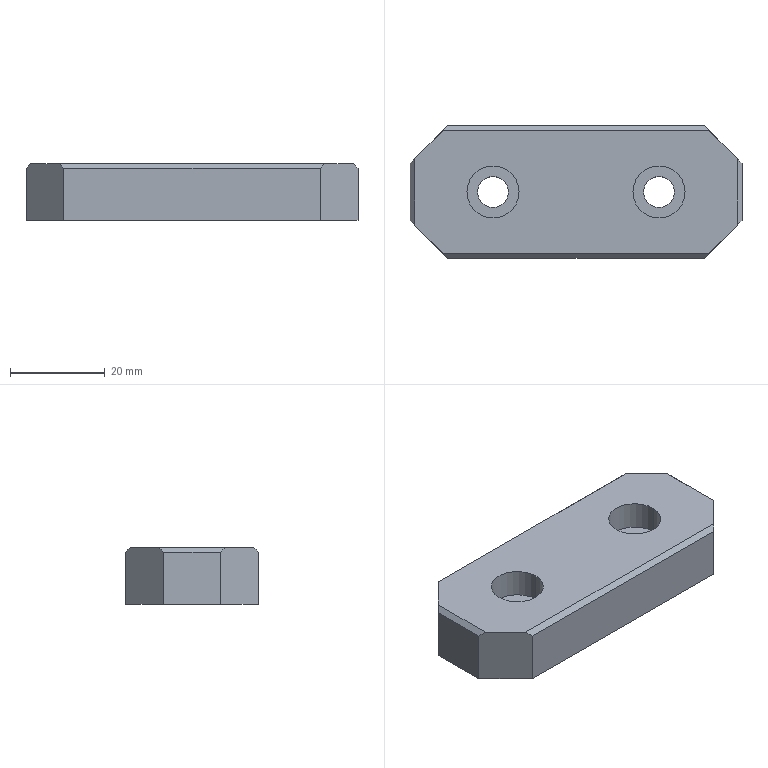Component | SolidWorks | DZ.KX.203-TC1505-30-09-01-05-05-1 | 1 solid | 24 faces | box 70 x 28 x 12 mm | volume 20378 mm3 | plane 16 | cylinder 8 | commonest cylinder face diameters 11 x4 6.5 x4 | material Plain Carbon Steel
build123d program:
from build123d import *

# Parameters (mm, degrees)
SKETCH1_W                                         = 70
SKETCH1_H                                         = 28
BOSS_EXTRUDE1_DEPTH                               = 12
HOLE_SIZE_ACCORDING_TO_HEXAGON_SOCKET_D           = 6.5
HOLE_SIZE_ACCORDING_TO_HEXAGON_SOCKET_CBORE_D     = 11
HOLE_SIZE_ACCORDING_TO_HEXAGON_SOCKET_CBORE_DEPTH = 6
CHAMFER2_SIZE                                     = 8
CHAMFER3_SIZE                                     = 1


with BuildPart() as part:
    # Sketch1 → Boss-Extrude1 (new body)
    with BuildSketch(Plane(origin=(0, 0, 0), x_dir=(0, 0, -1), z_dir=(1, 0, 0))):
        Rectangle(SKETCH1_W, SKETCH1_H)
    extrude(amount=BOSS_EXTRUDE1_DEPTH)

    # Hole Size _according to_ Hexagon Socket (through all)
    with Locations(Plane.ZY):
        with Locations((-17.5, 0), (17.5, 0)):
            CounterBoreHole(HOLE_SIZE_ACCORDING_TO_HEXAGON_SOCKET_D / 2, HOLE_SIZE_ACCORDING_TO_HEXAGON_SOCKET_CBORE_D / 2, HOLE_SIZE_ACCORDING_TO_HEXAGON_SOCKET_CBORE_DEPTH)

    # Chamfer2
    chamfer2_edges = [part.edges().sort_by_distance(p)[0] for p in [
        (6, 14, 35),
        (6, 14, -35),
        (6, -14, -35),
        (6, -14, 35),
    ]]
    chamfer(chamfer2_edges, length=CHAMFER2_SIZE)

    # Chamfer3
    chamfer3_edges = [part.edges().sort_by_distance(p)[0] for p in [
        (0, 0, 35),
        (0, 14, 0),
        (0, 0, -35),
        (0, -14, 0),
    ]]
    chamfer(chamfer3_edges, length=CHAMFER3_SIZE)


solid = part.part

# Placed as in the assembly
solid = solid.moved(Location((294.5, -610.807, 225.06), (0, 90, 0)))
STEP:
#1=COLOUR_RGB('',0.7922,0.8196,0.9333);
#2=FILL_AREA_STYLE_COLOUR('',#1);
#3=FILL_AREA_STYLE('',(#2));
#4=SURFACE_STYLE_FILL_AREA(#3);
#5=SURFACE_SIDE_STYLE('',(#4));
#6=SURFACE_STYLE_USAGE(.BOTH.,#5);
#7=PRESENTATION_STYLE_ASSIGNMENT((#6));
#8=CARTESIAN_POINT('',(10.689,-24.048,8.624));
#9=VERTEX_POINT('',#8);
#10=CARTESIAN_POINT('',(11.122,-24.048,8.624));
#11=VERTEX_POINT('',#10);
#12=CARTESIAN_POINT('',(10.906,-24.048,8.624));
#13=DIRECTION('',(0.,-0.,1.));
#14=DIRECTION('',(1.,0.,0.));
#15=AXIS2_PLACEMENT_3D('',#12,#13,#14);
#16=CIRCLE('',#15,0.2165);
#17=EDGE_CURVE('',#9,#11,#16,.T.);
#18=ORIENTED_EDGE('',*,*,#17,.F.);
#19=CARTESIAN_POINT('',(10.689,-24.048,8.861));
#20=VERTEX_POINT('',#19);
#21=CARTESIAN_POINT('',(10.689,-24.048,8.861));
#22=DIRECTION('',(0.,-0.,1.));
#23=VECTOR('',#22,39.37);
#24=LINE('',#21,#23);
#25=EDGE_CURVE('',#9,#20,#24,.T.);
#26=ORIENTED_EDGE('',*,*,#25,.T.);
#27=CARTESIAN_POINT('',(11.122,-24.048,8.861));
#28=VERTEX_POINT('',#27);
#29=CARTESIAN_POINT('',(10.906,-24.048,8.861));
#30=DIRECTION('',(0.,-0.,1.));
#31=DIRECTION('',(1.,0.,0.));
#32=AXIS2_PLACEMENT_3D('',#29,#30,#31);
#33=CIRCLE('',#32,0.2165);
#34=EDGE_CURVE('',#20,#28,#33,.T.);
#35=ORIENTED_EDGE('',*,*,#34,.T.);
#36=CARTESIAN_POINT('',(11.122,-24.048,8.861));
#37=DIRECTION('',(0.,-0.,1.));
#38=VECTOR('',#37,39.37);
#39=LINE('',#36,#38);
#40=EDGE_CURVE('',#11,#28,#39,.T.);
#41=ORIENTED_EDGE('',*,*,#40,.F.);
#42=EDGE_LOOP('',(#18,#26,#35,#41));
#43=FACE_OUTER_BOUND('',#42,.T.);
#44=CARTESIAN_POINT('',(10.906,-24.048,8.861));
#45=DIRECTION('',(0.,-0.,1.));
#46=DIRECTION('',(1.,0.,0.));
#47=AXIS2_PLACEMENT_3D('',#44,#45,#46);
#48=CYLINDRICAL_SURFACE('',#47,0.2165);
#49=ADVANCED_FACE('',(#43),#48,.F.);
#50=CARTESIAN_POINT('',(10.778,-24.048,8.388));
#51=VERTEX_POINT('',#50);
#52=CARTESIAN_POINT('',(11.033,-24.048,8.388));
#53=VERTEX_POINT('',#52);
#54=CARTESIAN_POINT('',(10.906,-24.048,8.388));
#55=DIRECTION('',(0.,-0.,1.));
#56=DIRECTION('',(1.,0.,0.));
#57=AXIS2_PLACEMENT_3D('',#54,#55,#56);
#58=CIRCLE('',#57,0.128);
#59=EDGE_CURVE('',#51,#53,#58,.T.);
#60=ORIENTED_EDGE('',*,*,#59,.F.);
#61=CARTESIAN_POINT('',(10.778,-24.048,8.624));
#62=VERTEX_POINT('',#61);
#63=CARTESIAN_POINT('',(10.778,-24.048,8.861));
#64=DIRECTION('',(0.,-0.,1.));
#65=VECTOR('',#64,39.37);
#66=LINE('',#63,#65);
#67=EDGE_CURVE('',#51,#62,#66,.T.);
#68=ORIENTED_EDGE('',*,*,#67,.T.);
#69=CARTESIAN_POINT('',(11.033,-24.048,8.624));
#70=VERTEX_POINT('',#69);
#71=CARTESIAN_POINT('',(10.906,-24.048,8.624));
#72=DIRECTION('',(0.,-0.,1.));
#73=DIRECTION('',(1.,0.,0.));
#74=AXIS2_PLACEMENT_3D('',#71,#72,#73);
#75=CIRCLE('',#74,0.128);
#76=EDGE_CURVE('',#62,#70,#75,.T.);
#77=ORIENTED_EDGE('',*,*,#76,.T.);
#78=CARTESIAN_POINT('',(11.033,-24.048,8.861));
#79=DIRECTION('',(0.,-0.,1.));
#80=VECTOR('',#79,39.37);
#81=LINE('',#78,#80);
#82=EDGE_CURVE('',#53,#70,#81,.T.);
#83=ORIENTED_EDGE('',*,*,#82,.F.);
#84=EDGE_LOOP('',(#60,#68,#77,#83));
#85=FACE_OUTER_BOUND('',#84,.T.);
#86=CARTESIAN_POINT('',(10.906,-24.048,8.861));
#87=DIRECTION('',(0.,-0.,1.));
#88=DIRECTION('',(1.,0.,0.));
#89=AXIS2_PLACEMENT_3D('',#86,#87,#88);
#90=CYLINDRICAL_SURFACE('',#89,0.128);
#91=ADVANCED_FACE('',(#85),#90,.F.);
#92=CARTESIAN_POINT('',(12.067,-24.048,8.624));
#93=VERTEX_POINT('',#92);
#94=CARTESIAN_POINT('',(12.5,-24.048,8.624));
#95=VERTEX_POINT('',#94);
#96=CARTESIAN_POINT('',(12.283,-24.048,8.624));
#97=DIRECTION('',(0.,-0.,1.));
#98=DIRECTION('',(1.,0.,0.));
#99=AXIS2_PLACEMENT_3D('',#96,#97,#98);
#100=CIRCLE('',#99,0.2165);
#101=EDGE_CURVE('',#93,#95,#100,.T.);
#102=ORIENTED_EDGE('',*,*,#101,.F.);
#103=CARTESIAN_POINT('',(12.067,-24.048,8.861));
#104=VERTEX_POINT('',#103);
#105=CARTESIAN_POINT('',(12.067,-24.048,8.861));
#106=DIRECTION('',(0.,-0.,1.));
#107=VECTOR('',#106,39.37);
#108=LINE('',#105,#107);
#109=EDGE_CURVE('',#93,#104,#108,.T.);
#110=ORIENTED_EDGE('',*,*,#109,.T.);
#111=CARTESIAN_POINT('',(12.5,-24.048,8.861));
#112=VERTEX_POINT('',#111);
#113=CARTESIAN_POINT('',(12.283,-24.048,8.861));
#114=DIRECTION('',(0.,-0.,1.));
#115=DIRECTION('',(1.,0.,0.));
#116=AXIS2_PLACEMENT_3D('',#113,#114,#115);
#117=CIRCLE('',#116,0.2165);
#118=EDGE_CURVE('',#104,#112,#117,.T.);
#119=ORIENTED_EDGE('',*,*,#118,.T.);
#120=CARTESIAN_POINT('',(12.5,-24.048,8.861));
#121=DIRECTION('',(0.,-0.,1.));
#122=VECTOR('',#121,39.37);
#123=LINE('',#120,#122);
#124=EDGE_CURVE('',#95,#112,#123,.T.);
#125=ORIENTED_EDGE('',*,*,#124,.F.);
#126=EDGE_LOOP('',(#102,#110,#119,#125));
#127=FACE_OUTER_BOUND('',#126,.T.);
#128=CARTESIAN_POINT('',(12.283,-24.048,8.861));
#129=DIRECTION('',(0.,-0.,1.));
#130=DIRECTION('',(1.,0.,0.));
#131=AXIS2_PLACEMENT_3D('',#128,#129,#130);
#132=CYLINDRICAL_SURFACE('',#131,0.2165);
#133=ADVANCED_FACE('',(#127),#132,.F.);
#134=CARTESIAN_POINT('',(12.156,-24.048,8.388));
#135=VERTEX_POINT('',#134);
#136=CARTESIAN_POINT('',(12.411,-24.048,8.388));
#137=VERTEX_POINT('',#136);
#138=CARTESIAN_POINT('',(12.283,-24.048,8.388));
#139=DIRECTION('',(0.,-0.,1.));
#140=DIRECTION('',(1.,0.,0.));
#141=AXIS2_PLACEMENT_3D('',#138,#139,#140);
#142=CIRCLE('',#141,0.128);
#143=EDGE_CURVE('',#135,#137,#142,.T.);
#144=ORIENTED_EDGE('',*,*,#143,.F.);
#145=CARTESIAN_POINT('',(12.156,-24.048,8.624));
#146=VERTEX_POINT('',#145);
#147=CARTESIAN_POINT('',(12.156,-24.048,8.861));
#148=DIRECTION('',(0.,-0.,1.));
#149=VECTOR('',#148,39.37);
#150=LINE('',#147,#149);
#151=EDGE_CURVE('',#135,#146,#150,.T.);
#152=ORIENTED_EDGE('',*,*,#151,.T.);
#153=CARTESIAN_POINT('',(12.411,-24.048,8.624));
#154=VERTEX_POINT('',#153);
#155=CARTESIAN_POINT('',(12.283,-24.048,8.624));
#156=DIRECTION('',(0.,-0.,1.));
#157=DIRECTION('',(1.,0.,0.));
#158=AXIS2_PLACEMENT_3D('',#155,#156,#157);
#159=CIRCLE('',#158,0.128);
#160=EDGE_CURVE('',#146,#154,#159,.T.);
#161=ORIENTED_EDGE('',*,*,#160,.T.);
#162=CARTESIAN_POINT('',(12.411,-24.048,8.861));
#163=DIRECTION('',(0.,-0.,1.));
#164=VECTOR('',#163,39.37);
#165=LINE('',#162,#164);
#166=EDGE_CURVE('',#137,#154,#165,.T.);
#167=ORIENTED_EDGE('',*,*,#166,.F.);
#168=EDGE_LOOP('',(#144,#152,#161,#167));
#169=FACE_OUTER_BOUND('',#168,.T.);
#170=CARTESIAN_POINT('',(12.283,-24.048,8.861));
#171=DIRECTION('',(0.,-0.,1.));
#172=DIRECTION('',(1.,0.,0.));
#173=AXIS2_PLACEMENT_3D('',#170,#171,#172);
#174=CYLINDRICAL_SURFACE('',#173,0.128);
#175=ADVANCED_FACE('',(#169),#174,.F.);
#176=CARTESIAN_POINT('',(12.972,-23.811,8.388));
#177=VERTEX_POINT('',#176);
#178=CARTESIAN_POINT('',(12.972,-23.811,8.821));
#179=VERTEX_POINT('',#178);
#180=CARTESIAN_POINT('',(12.972,-23.811,8.388));
#181=DIRECTION('',(0.,-0.,1.));
#182=VECTOR('',#181,39.37);
#183=LINE('',#180,#182);
#184=EDGE_CURVE('',#177,#179,#183,.T.);
#185=ORIENTED_EDGE('',*,*,#184,.T.);
#186=CARTESIAN_POINT('',(12.972,-24.284,8.821));
#187=VERTEX_POINT('',#186);
#188=CARTESIAN_POINT('',(12.972,-24.599,8.821));
#189=DIRECTION('',(-0.,-1.,-0.));
#190=VECTOR('',#189,39.37);
#191=LINE('',#188,#190);
#192=EDGE_CURVE('',#179,#187,#191,.T.);
#193=ORIENTED_EDGE('',*,*,#192,.T.);
#194=CARTESIAN_POINT('',(12.972,-24.284,8.388));
#195=VERTEX_POINT('',#194);
#196=CARTESIAN_POINT('',(12.972,-24.284,8.388));
#197=DIRECTION('',(-0.,0.,-1.));
#198=VECTOR('',#197,39.37);
#199=LINE('',#196,#198);
#200=EDGE_CURVE('',#187,#195,#199,.T.);
#201=ORIENTED_EDGE('',*,*,#200,.T.);
#202=CARTESIAN_POINT('',(12.972,-24.599,8.388));
#203=DIRECTION('',(-0.,-1.,-0.));
#204=VECTOR('',#203,39.37);
#205=LINE('',#202,#204);
#206=EDGE_CURVE('',#177,#195,#205,.T.);
#207=ORIENTED_EDGE('',*,*,#206,.F.);
#208=EDGE_LOOP('',(#185,#193,#201,#207));
#209=FACE_OUTER_BOUND('',#208,.T.);
#210=CARTESIAN_POINT('',(12.972,-24.599,8.388));
#211=DIRECTION('',(-1.,0.,0.));
#212=DIRECTION('',(0.,-0.,1.));
#213=AXIS2_PLACEMENT_3D('',#210,#211,#212);
#214=PLANE('',#213);
#215=ADVANCED_FACE('',(#209),#214,.F.);
#216=CARTESIAN_POINT('',(12.657,-24.599,8.388));
#217=VERTEX_POINT('',#216);
#218=CARTESIAN_POINT('',(12.657,-24.599,8.821));
#219=VERTEX_POINT('',#218);
#220=CARTESIAN_POINT('',(12.657,-24.599,8.388));
#221=DIRECTION('',(0.,-0.,1.));
#222=VECTOR('',#221,39.37);
#223=LINE('',#220,#222);
#224=EDGE_CURVE('',#217,#219,#223,.T.);
#225=ORIENTED_EDGE('',*,*,#224,.T.);
#226=CARTESIAN_POINT('',(10.531,-24.599,8.821));
#227=VERTEX_POINT('',#226);
#228=CARTESIAN_POINT('',(10.217,-24.599,8.821));
#229=DIRECTION('',(-1.,0.,0.));
#230=VECTOR('',#229,39.37);
#231=LINE('',#228,#230);
#232=EDGE_CURVE('',#219,#227,#231,.T.);
#233=ORIENTED_EDGE('',*,*,#232,.T.);
#234=CARTESIAN_POINT('',(10.531,-24.599,8.388));
#235=VERTEX_POINT('',#234);
#236=CARTESIAN_POINT('',(10.531,-24.599,8.388));
#237=DIRECTION('',(-0.,0.,-1.));
#238=VECTOR('',#237,39.37);
#239=LINE('',#236,#238);
#240=EDGE_CURVE('',#227,#235,#239,.T.);
#241=ORIENTED_EDGE('',*,*,#240,.T.);
#242=CARTESIAN_POINT('',(10.217,-24.599,8.388));
#243=DIRECTION('',(-1.,0.,0.));
#244=VECTOR('',#243,39.37);
#245=LINE('',#242,#244);
#246=EDGE_CURVE('',#217,#235,#245,.T.);
#247=ORIENTED_EDGE('',*,*,#246,.F.);
#248=EDGE_LOOP('',(#225,#233,#241,#247));
#249=FACE_OUTER_BOUND('',#248,.T.);
#250=CARTESIAN_POINT('',(10.217,-24.599,8.388));
#251=DIRECTION('',(0.,1.,0.));
#252=DIRECTION('',(1.,-0.,-0.));
#253=AXIS2_PLACEMENT_3D('',#250,#251,#252);
#254=PLANE('',#253);
#255=ADVANCED_FACE('',(#249),#254,.F.);
#256=CARTESIAN_POINT('',(10.217,-24.284,8.388));
#257=VERTEX_POINT('',#256);
#258=CARTESIAN_POINT('',(10.217,-24.284,8.821));
#259=VERTEX_POINT('',#258);
#260=CARTESIAN_POINT('',(10.217,-24.284,8.388));
#261=DIRECTION('',(0.,-0.,1.));
#262=VECTOR('',#261,39.37);
#263=LINE('',#260,#262);
#264=EDGE_CURVE('',#257,#259,#263,.T.);
#265=ORIENTED_EDGE('',*,*,#264,.T.);
#266=CARTESIAN_POINT('',(10.217,-23.811,8.821));
#267=VERTEX_POINT('',#266);
#268=CARTESIAN_POINT('',(10.217,-24.599,8.821));
#269=DIRECTION('',(0.,1.,0.));
#270=VECTOR('',#269,39.37);
#271=LINE('',#268,#270);
#272=EDGE_CURVE('',#259,#267,#271,.T.);
#273=ORIENTED_EDGE('',*,*,#272,.T.);
#274=CARTESIAN_POINT('',(10.217,-23.811,8.388));
#275=VERTEX_POINT('',#274);
#276=CARTESIAN_POINT('',(10.217,-23.811,8.388));
#277=DIRECTION('',(-0.,0.,-1.));
#278=VECTOR('',#277,39.37);
#279=LINE('',#276,#278);
#280=EDGE_CURVE('',#267,#275,#279,.T.);
#281=ORIENTED_EDGE('',*,*,#280,.T.);
#282=CARTESIAN_POINT('',(10.217,-24.599,8.388));
#283=DIRECTION('',(0.,1.,0.));
#284=VECTOR('',#283,39.37);
#285=LINE('',#282,#284);
#286=EDGE_CURVE('',#257,#275,#285,.T.);
#287=ORIENTED_EDGE('',*,*,#286,.F.);
#288=EDGE_LOOP('',(#265,#273,#281,#287));
#289=FACE_OUTER_BOUND('',#288,.T.);
#290=CARTESIAN_POINT('',(10.217,-24.599,8.388));
#291=DIRECTION('',(1.,-0.,-0.));
#292=DIRECTION('',(-0.,0.,-1.));
#293=AXIS2_PLACEMENT_3D('',#290,#291,#292);
#294=PLANE('',#293);
#295=ADVANCED_FACE('',(#289),#294,.F.);
#296=CARTESIAN_POINT('',(10.531,-23.496,8.388));
#297=VERTEX_POINT('',#296);
#298=CARTESIAN_POINT('',(10.531,-23.496,8.821));
#299=VERTEX_POINT('',#298);
#300=CARTESIAN_POINT('',(10.531,-23.496,8.388));
#301=DIRECTION('',(0.,-0.,1.));
#302=VECTOR('',#301,39.37);
#303=LINE('',#300,#302);
#304=EDGE_CURVE('',#297,#299,#303,.T.);
#305=ORIENTED_EDGE('',*,*,#304,.T.);
#306=CARTESIAN_POINT('',(12.657,-23.496,8.821));
#307=VERTEX_POINT('',#306);
#308=CARTESIAN_POINT('',(10.217,-23.496,8.821));
#309=DIRECTION('',(1.,-0.,-0.));
#310=VECTOR('',#309,39.37);
#311=LINE('',#308,#310);
#312=EDGE_CURVE('',#299,#307,#311,.T.);
#313=ORIENTED_EDGE('',*,*,#312,.T.);
#314=CARTESIAN_POINT('',(12.657,-23.496,8.388));
#315=VERTEX_POINT('',#314);
#316=CARTESIAN_POINT('',(12.657,-23.496,8.388));
#317=DIRECTION('',(-0.,0.,-1.));
#318=VECTOR('',#317,39.37);
#319=LINE('',#316,#318);
#320=EDGE_CURVE('',#307,#315,#319,.T.);
#321=ORIENTED_EDGE('',*,*,#320,.T.);
#322=CARTESIAN_POINT('',(10.217,-23.496,8.388));
#323=DIRECTION('',(1.,-0.,-0.));
#324=VECTOR('',#323,39.37);
#325=LINE('',#322,#324);
#326=EDGE_CURVE('',#297,#315,#325,.T.);
#327=ORIENTED_EDGE('',*,*,#326,.F.);
#328=EDGE_LOOP('',(#305,#313,#321,#327));
#329=FACE_OUTER_BOUND('',#328,.T.);
#330=CARTESIAN_POINT('',(10.217,-23.496,8.388));
#331=DIRECTION('',(-0.,-1.,-0.));
#332=DIRECTION('',(-1.,0.,0.));
#333=AXIS2_PLACEMENT_3D('',#330,#331,#332);
#334=PLANE('',#333);
#335=ADVANCED_FACE('',(#329),#334,.F.);
#336=CARTESIAN_POINT('',(10.906,-24.048,8.388));
#337=DIRECTION('',(0.,-0.,1.));
#338=DIRECTION('',(1.,0.,0.));
#339=AXIS2_PLACEMENT_3D('',#336,#337,#338);
#340=CIRCLE('',#339,0.128);
#341=EDGE_CURVE('',#53,#51,#340,.T.);
#342=ORIENTED_EDGE('',*,*,#341,.T.);
#343=ORIENTED_EDGE('',*,*,#59,.T.);
#344=EDGE_LOOP('',(#342,#343));
#345=FACE_BOUND('',#344,.T.);
#346=CARTESIAN_POINT('',(12.283,-24.048,8.388));
#347=DIRECTION('',(0.,-0.,1.));
#348=DIRECTION('',(1.,0.,0.));
#349=AXIS2_PLACEMENT_3D('',#346,#347,#348);
#350=CIRCLE('',#349,0.128);
#351=EDGE_CURVE('',#137,#135,#350,.T.);
#352=ORIENTED_EDGE('',*,*,#351,.T.);
#353=ORIENTED_EDGE('',*,*,#143,.T.);
#354=EDGE_LOOP('',(#352,#353));
#355=FACE_BOUND('',#354,.T.);
#356=ORIENTED_EDGE('',*,*,#326,.T.);
#357=CARTESIAN_POINT('',(12.402,-23.24,8.388));
#358=DIRECTION('',(0.7071,-0.7071,-0.));
#359=VECTOR('',#358,39.37);
#360=LINE('',#357,#359);
#361=EDGE_CURVE('',#315,#177,#360,.T.);
#362=ORIENTED_EDGE('',*,*,#361,.T.);
#363=ORIENTED_EDGE('',*,*,#206,.T.);
#364=CARTESIAN_POINT('',(12.402,-24.855,8.388));
#365=DIRECTION('',(-0.7071,-0.7071,-0.));
#366=VECTOR('',#365,39.37);
#367=LINE('',#364,#366);
#368=EDGE_CURVE('',#195,#217,#367,.T.);
#369=ORIENTED_EDGE('',*,*,#368,.T.);
#370=ORIENTED_EDGE('',*,*,#246,.T.);
#371=CARTESIAN_POINT('',(10.787,-24.855,8.388));
#372=DIRECTION('',(-0.7071,0.7071,0.));
#373=VECTOR('',#372,39.37);
#374=LINE('',#371,#373);
#375=EDGE_CURVE('',#235,#257,#374,.T.);
#376=ORIENTED_EDGE('',*,*,#375,.T.);
#377=ORIENTED_EDGE('',*,*,#286,.T.);
#378=CARTESIAN_POINT('',(10.787,-23.24,8.388));
#379=DIRECTION('',(0.7071,0.7071,0.));
#380=VECTOR('',#379,39.37);
#381=LINE('',#378,#380);
#382=EDGE_CURVE('',#275,#297,#381,.T.);
#383=ORIENTED_EDGE('',*,*,#382,.T.);
#384=EDGE_LOOP('',(#356,#362,#363,#369,#370,#376,#377,#383));
#385=FACE_OUTER_BOUND('',#384,.T.);
#386=CARTESIAN_POINT('',(11.594,-24.048,8.388));
#387=DIRECTION('',(-0.,0.,-1.));
#388=DIRECTION('',(-1.,0.,0.));
#389=AXIS2_PLACEMENT_3D('',#386,#387,#388);
#390=PLANE('',#389);
#391=ADVANCED_FACE('',(#345,#355,#385),#390,.T.);
#392=CARTESIAN_POINT('',(10.906,-24.048,8.861));
#393=DIRECTION('',(0.,-0.,1.));
#394=DIRECTION('',(1.,0.,0.));
#395=AXIS2_PLACEMENT_3D('',#392,#393,#394);
#396=CIRCLE('',#395,0.2165);
#397=EDGE_CURVE('',#28,#20,#396,.T.);
#398=ORIENTED_EDGE('',*,*,#397,.F.);
#399=ORIENTED_EDGE('',*,*,#34,.F.);
#400=EDGE_LOOP('',(#398,#399));
#401=FACE_BOUND('',#400,.T.);
#402=CARTESIAN_POINT('',(12.283,-24.048,8.861));
#403=DIRECTION('',(0.,-0.,1.));
#404=DIRECTION('',(1.,0.,0.));
#405=AXIS2_PLACEMENT_3D('',#402,#403,#404);
#406=CIRCLE('',#405,0.2165);
#407=EDGE_CURVE('',#112,#104,#406,.T.);
#408=ORIENTED_EDGE('',*,*,#407,.F.);
#409=ORIENTED_EDGE('',*,*,#118,.F.);
#410=EDGE_LOOP('',(#408,#409));
#411=FACE_BOUND('',#410,.T.);
#412=CARTESIAN_POINT('',(12.933,-23.772,8.861));
#413=VERTEX_POINT('',#412);
#414=CARTESIAN_POINT('',(12.697,-23.536,8.861));
#415=VERTEX_POINT('',#414);
#416=CARTESIAN_POINT('',(12.972,-23.811,8.861));
#417=DIRECTION('',(-0.7071,0.7071,0.));
#418=VECTOR('',#417,39.37);
#419=LINE('',#416,#418);
#420=EDGE_CURVE('',#413,#415,#419,.T.);
#421=ORIENTED_EDGE('',*,*,#420,.T.);
#422=CARTESIAN_POINT('',(10.492,-23.536,8.861));
#423=VERTEX_POINT('',#422);
#424=CARTESIAN_POINT('',(11.594,-23.536,8.861));
#425=DIRECTION('',(-1.,0.,0.));
#426=VECTOR('',#425,39.37);
#427=LINE('',#424,#426);
#428=EDGE_CURVE('',#415,#423,#427,.T.);
#429=ORIENTED_EDGE('',*,*,#428,.T.);
#430=CARTESIAN_POINT('',(10.256,-23.772,8.861));
#431=VERTEX_POINT('',#430);
#432=CARTESIAN_POINT('',(10.531,-23.496,8.861));
#433=DIRECTION('',(-0.7071,-0.7071,-0.));
#434=VECTOR('',#433,39.37);
#435=LINE('',#432,#434);
#436=EDGE_CURVE('',#423,#431,#435,.T.);
#437=ORIENTED_EDGE('',*,*,#436,.T.);
#438=CARTESIAN_POINT('',(10.256,-24.323,8.861));
#439=VERTEX_POINT('',#438);
#440=CARTESIAN_POINT('',(10.256,-24.048,8.861));
#441=DIRECTION('',(-0.,-1.,-0.));
#442=VECTOR('',#441,39.37);
#443=LINE('',#440,#442);
#444=EDGE_CURVE('',#431,#439,#443,.T.);
#445=ORIENTED_EDGE('',*,*,#444,.T.);
#446=CARTESIAN_POINT('',(10.492,-24.559,8.861));
#447=VERTEX_POINT('',#446);
#448=CARTESIAN_POINT('',(10.217,-24.284,8.861));
#449=DIRECTION('',(0.7071,-0.7071,-0.));
#450=VECTOR('',#449,39.37);
#451=LINE('',#448,#450);
#452=EDGE_CURVE('',#439,#447,#451,.T.);
#453=ORIENTED_EDGE('',*,*,#452,.T.);
#454=CARTESIAN_POINT('',(12.697,-24.559,8.861));
#455=VERTEX_POINT('',#454);
#456=CARTESIAN_POINT('',(11.594,-24.559,8.861));
#457=DIRECTION('',(1.,-0.,-0.));
#458=VECTOR('',#457,39.37);
#459=LINE('',#456,#458);
#460=EDGE_CURVE('',#447,#455,#459,.T.);
#461=ORIENTED_EDGE('',*,*,#460,.T.);
#462=CARTESIAN_POINT('',(12.933,-24.323,8.861));
#463=VERTEX_POINT('',#462);
#464=CARTESIAN_POINT('',(12.657,-24.599,8.861));
#465=DIRECTION('',(0.7071,0.7071,0.));
#466=VECTOR('',#465,39.37);
#467=LINE('',#464,#466);
#468=EDGE_CURVE('',#455,#463,#467,.T.);
#469=ORIENTED_EDGE('',*,*,#468,.T.);
#470=CARTESIAN_POINT('',(12.933,-24.048,8.861));
#471=DIRECTION('',(0.,1.,0.));
#472=VECTOR('',#471,39.37);
#473=LINE('',#470,#472);
#474=EDGE_CURVE('',#463,#413,#473,.T.);
#475=ORIENTED_EDGE('',*,*,#474,.T.);
#476=EDGE_LOOP('',(#421,#429,#437,#445,#453,#461,#469,#475));
#477=FACE_OUTER_BOUND('',#476,.T.);
#478=CARTESIAN_POINT('',(11.594,-24.048,8.861));
#479=DIRECTION('',(-0.,0.,-1.));
#480=DIRECTION('',(-1.,0.,0.));
#481=AXIS2_PLACEMENT_3D('',#478,#479,#480);
#482=PLANE('',#481);
#483=ADVANCED_FACE('',(#401,#411,#477),#482,.F.);
#484=ORIENTED_EDGE('',*,*,#151,.F.);
#485=ORIENTED_EDGE('',*,*,#351,.F.);
#486=ORIENTED_EDGE('',*,*,#166,.T.);
#487=CARTESIAN_POINT('',(12.283,-24.048,8.624));
#488=DIRECTION('',(0.,-0.,1.));
#489=DIRECTION('',(1.,0.,0.));
#490=AXIS2_PLACEMENT_3D('',#487,#488,#489);
#491=CIRCLE('',#490,0.128);
#492=EDGE_CURVE('',#154,#146,#491,.T.);
#493=ORIENTED_EDGE('',*,*,#492,.T.);
#494=EDGE_LOOP('',(#484,#485,#486,#493));
#495=FACE_OUTER_BOUND('',#494,.T.);
#496=CARTESIAN_POINT('',(12.283,-24.048,8.861));
#497=DIRECTION('',(0.,-0.,1.));
#498=DIRECTION('',(1.,0.,0.));
#499=AXIS2_PLACEMENT_3D('',#496,#497,#498);
#500=CYLINDRICAL_SURFACE('',#499,0.128);
#501=ADVANCED_FACE('',(#495),#500,.F.);
#502=ORIENTED_EDGE('',*,*,#492,.F.);
#503=ORIENTED_EDGE('',*,*,#160,.F.);
#504=EDGE_LOOP('',(#502,#503));
#505=FACE_BOUND('',#504,.T.);
#506=CARTESIAN_POINT('',(12.283,-24.048,8.624));
#507=DIRECTION('',(0.,-0.,1.));
#508=DIRECTION('',(1.,0.,0.));
#509=AXIS2_PLACEMENT_3D('',#506,#507,#508);
#510=CIRCLE('',#509,0.2165);
#511=EDGE_CURVE('',#95,#93,#510,.T.);
#512=ORIENTED_EDGE('',*,*,#511,.T.);
#513=ORIENTED_EDGE('',*,*,#101,.T.);
#514=EDGE_LOOP('',(#512,#513));
#515=FACE_OUTER_BOUND('',#514,.T.);
#516=CARTESIAN_POINT('',(12.283,-23.92,8.624));
#517=DIRECTION('',(-0.,0.,-1.));
#518=DIRECTION('',(-1.,0.,0.));
#519=AXIS2_PLACEMENT_3D('',#516,#517,#518);
#520=PLANE('',#519);
#521=ADVANCED_FACE('',(#505,#515),#520,.F.);
#522=ORIENTED_EDGE('',*,*,#109,.F.);
#523=ORIENTED_EDGE('',*,*,#511,.F.);
#524=ORIENTED_EDGE('',*,*,#124,.T.);
#525=ORIENTED_EDGE('',*,*,#407,.T.);
#526=EDGE_LOOP('',(#522,#523,#524,#525));
#527=FACE_OUTER_BOUND('',#526,.T.);
#528=CARTESIAN_POINT('',(12.283,-24.048,8.861));
#529=DIRECTION('',(0.,-0.,1.));
#530=DIRECTION('',(1.,0.,0.));
#531=AXIS2_PLACEMENT_3D('',#528,#529,#530);
#532=CYLINDRICAL_SURFACE('',#531,0.2165);
#533=ADVANCED_FACE('',(#527),#532,.F.);
#534=ORIENTED_EDGE('',*,*,#67,.F.);
#535=ORIENTED_EDGE('',*,*,#341,.F.);
#536=ORIENTED_EDGE('',*,*,#82,.T.);
#537=CARTESIAN_POINT('',(10.906,-24.048,8.624));
#538=DIRECTION('',(0.,-0.,1.));
#539=DIRECTION('',(1.,0.,0.));
#540=AXIS2_PLACEMENT_3D('',#537,#538,#539);
#541=CIRCLE('',#540,0.128);
#542=EDGE_CURVE('',#70,#62,#541,.T.);
#543=ORIENTED_EDGE('',*,*,#542,.T.);
#544=EDGE_LOOP('',(#534,#535,#536,#543));
#545=FACE_OUTER_BOUND('',#544,.T.);
#546=CARTESIAN_POINT('',(10.906,-24.048,8.861));
#547=DIRECTION('',(0.,-0.,1.));
#548=DIRECTION('',(1.,0.,0.));
#549=AXIS2_PLACEMENT_3D('',#546,#547,#548);
#550=CYLINDRICAL_SURFACE('',#549,0.128);
#551=ADVANCED_FACE('',(#545),#550,.F.);
#552=ORIENTED_EDGE('',*,*,#542,.F.);
#553=ORIENTED_EDGE('',*,*,#76,.F.);
#554=EDGE_LOOP('',(#552,#553));
#555=FACE_BOUND('',#554,.T.);
#556=CARTESIAN_POINT('',(10.906,-24.048,8.624));
#557=DIRECTION('',(0.,-0.,1.));
#558=DIRECTION('',(1.,0.,0.));
#559=AXIS2_PLACEMENT_3D('',#556,#557,#558);
#560=CIRCLE('',#559,0.2165);
#561=EDGE_CURVE('',#11,#9,#560,.T.);
#562=ORIENTED_EDGE('',*,*,#561,.T.);
#563=ORIENTED_EDGE('',*,*,#17,.T.);
#564=EDGE_LOOP('',(#562,#563));
#565=FACE_OUTER_BOUND('',#564,.T.);
#566=CARTESIAN_POINT('',(10.906,-23.92,8.624));
#567=DIRECTION('',(-0.,0.,-1.));
#568=DIRECTION('',(-1.,0.,0.));
#569=AXIS2_PLACEMENT_3D('',#566,#567,#568);
#570=PLANE('',#569);
#571=ADVANCED_FACE('',(#555,#565),#570,.F.);
#572=ORIENTED_EDGE('',*,*,#25,.F.);
#573=ORIENTED_EDGE('',*,*,#561,.F.);
#574=ORIENTED_EDGE('',*,*,#40,.T.);
#575=ORIENTED_EDGE('',*,*,#397,.T.);
#576=EDGE_LOOP('',(#572,#573,#574,#575));
#577=FACE_OUTER_BOUND('',#576,.T.);
#578=CARTESIAN_POINT('',(10.906,-24.048,8.861));
#579=DIRECTION('',(0.,-0.,1.));
#580=DIRECTION('',(1.,0.,0.));
#581=AXIS2_PLACEMENT_3D('',#578,#579,#580);
#582=CYLINDRICAL_SURFACE('',#581,0.2165);
#583=ADVANCED_FACE('',(#577),#582,.F.);
#584=ORIENTED_EDGE('',*,*,#320,.F.);
#585=CARTESIAN_POINT('',(12.723,-23.562,8.887));
#586=DIRECTION('',(0.5774,-0.5774,0.5774));
#587=VECTOR('',#586,39.37);
#588=LINE('',#585,#587);
#589=EDGE_CURVE('',#307,#415,#588,.T.);
#590=ORIENTED_EDGE('',*,*,#589,.T.);
#591=ORIENTED_EDGE('',*,*,#420,.F.);
#592=CARTESIAN_POINT('',(13.117,-23.956,8.677));
#593=DIRECTION('',(0.5774,-0.5774,-0.5774));
#594=VECTOR('',#593,39.37);
#595=LINE('',#592,#594);
#596=EDGE_CURVE('',#413,#179,#595,.T.);
#597=ORIENTED_EDGE('',*,*,#596,.T.);
#598=ORIENTED_EDGE('',*,*,#184,.F.);
#599=ORIENTED_EDGE('',*,*,#361,.F.);
#600=EDGE_LOOP('',(#584,#590,#591,#597,#598,#599));
#601=FACE_OUTER_BOUND('',#600,.T.);
#602=CARTESIAN_POINT('',(12.972,-23.811,8.388));
#603=DIRECTION('',(-0.7071,-0.7071,-0.));
#604=DIRECTION('',(0.,-0.,1.));
#605=AXIS2_PLACEMENT_3D('',#602,#603,#604);
#606=PLANE('',#605);
#607=ADVANCED_FACE('',(#601),#606,.F.);
#608=ORIENTED_EDGE('',*,*,#200,.F.);
#609=CARTESIAN_POINT('',(12.907,-24.349,8.887));
#610=DIRECTION('',(-0.5774,-0.5774,0.5774));
#611=VECTOR('',#610,39.37);
#612=LINE('',#609,#611);
#613=EDGE_CURVE('',#187,#463,#612,.T.);
#614=ORIENTED_EDGE('',*,*,#613,.T.);
#615=ORIENTED_EDGE('',*,*,#468,.F.);
#616=CARTESIAN_POINT('',(12.513,-24.743,8.677));
#617=DIRECTION('',(-0.5774,-0.5774,-0.5774));
#618=VECTOR('',#617,39.37);
#619=LINE('',#616,#618);
#620=EDGE_CURVE('',#455,#219,#619,.T.);
#621=ORIENTED_EDGE('',*,*,#620,.T.);
#622=ORIENTED_EDGE('',*,*,#224,.F.);
#623=ORIENTED_EDGE('',*,*,#368,.F.);
#624=EDGE_LOOP('',(#608,#614,#615,#621,#622,#623));
#625=FACE_OUTER_BOUND('',#624,.T.);
#626=CARTESIAN_POINT('',(12.657,-24.599,8.388));
#627=DIRECTION('',(-0.7071,0.7071,0.));
#628=DIRECTION('',(0.,-0.,1.));
#629=AXIS2_PLACEMENT_3D('',#626,#627,#628);
#630=PLANE('',#629);
#631=ADVANCED_FACE('',(#625),#630,.F.);
#632=ORIENTED_EDGE('',*,*,#436,.F.);
#633=CARTESIAN_POINT('',(10.676,-23.352,8.677));
#634=DIRECTION('',(0.5774,0.5774,-0.5774));
#635=VECTOR('',#634,39.37);
#636=LINE('',#633,#635);
#637=EDGE_CURVE('',#423,#299,#636,.T.);
#638=ORIENTED_EDGE('',*,*,#637,.T.);
#639=ORIENTED_EDGE('',*,*,#304,.F.);
#640=ORIENTED_EDGE('',*,*,#382,.F.);
#641=ORIENTED_EDGE('',*,*,#280,.F.);
#642=CARTESIAN_POINT('',(10.282,-23.746,8.887));
#643=DIRECTION('',(0.5774,0.5774,0.5774));
#644=VECTOR('',#643,39.37);
#645=LINE('',#642,#644);
#646=EDGE_CURVE('',#267,#431,#645,.T.);
#647=ORIENTED_EDGE('',*,*,#646,.T.);
#648=EDGE_LOOP('',(#632,#638,#639,#640,#641,#647));
#649=FACE_OUTER_BOUND('',#648,.T.);
#650=CARTESIAN_POINT('',(10.531,-23.496,8.388));
#651=DIRECTION('',(0.7071,-0.7071,-0.));
#652=DIRECTION('',(0.,-0.,1.));
#653=AXIS2_PLACEMENT_3D('',#650,#651,#652);
#654=PLANE('',#653);
#655=ADVANCED_FACE('',(#649),#654,.F.);
#656=ORIENTED_EDGE('',*,*,#452,.F.);
#657=CARTESIAN_POINT('',(10.072,-24.139,8.677));
#658=DIRECTION('',(-0.5774,0.5774,-0.5774));
#659=VECTOR('',#658,39.37);
#660=LINE('',#657,#659);
#661=EDGE_CURVE('',#439,#259,#660,.T.);
#662=ORIENTED_EDGE('',*,*,#661,.T.);
#663=ORIENTED_EDGE('',*,*,#264,.F.);
#664=ORIENTED_EDGE('',*,*,#375,.F.);
#665=ORIENTED_EDGE('',*,*,#240,.F.);
#666=CARTESIAN_POINT('',(10.466,-24.533,8.887));
#667=DIRECTION('',(-0.5774,0.5774,0.5774));
#668=VECTOR('',#667,39.37);
#669=LINE('',#666,#668);
#670=EDGE_CURVE('',#227,#447,#669,.T.);
#671=ORIENTED_EDGE('',*,*,#670,.T.);
#672=EDGE_LOOP('',(#656,#662,#663,#664,#665,#671));
#673=FACE_OUTER_BOUND('',#672,.T.);
#674=CARTESIAN_POINT('',(10.217,-24.284,8.388));
#675=DIRECTION('',(0.7071,0.7071,0.));
#676=DIRECTION('',(0.,-0.,1.));
#677=AXIS2_PLACEMENT_3D('',#674,#675,#676);
#678=PLANE('',#677);
#679=ADVANCED_FACE('',(#673),#678,.F.);
#680=ORIENTED_EDGE('',*,*,#637,.F.);
#681=ORIENTED_EDGE('',*,*,#428,.F.);
#682=ORIENTED_EDGE('',*,*,#589,.F.);
#683=ORIENTED_EDGE('',*,*,#312,.F.);
#684=EDGE_LOOP('',(#680,#681,#682,#683));
#685=FACE_OUTER_BOUND('',#684,.T.);
#686=CARTESIAN_POINT('',(10.217,-23.496,8.821));
#687=DIRECTION('',(-0.,-0.7071,-0.7071));
#688=DIRECTION('',(1.,-0.,-0.));
#689=AXIS2_PLACEMENT_3D('',#686,#687,#688);
#690=PLANE('',#689);
#691=ADVANCED_FACE('',(#685),#690,.F.);
#692=ORIENTED_EDGE('',*,*,#596,.F.);
#693=ORIENTED_EDGE('',*,*,#474,.F.);
#694=ORIENTED_EDGE('',*,*,#613,.F.);
#695=ORIENTED_EDGE('',*,*,#192,.F.);
#696=EDGE_LOOP('',(#692,#693,#694,#695));
#697=FACE_OUTER_BOUND('',#696,.T.);
#698=CARTESIAN_POINT('',(12.972,-24.599,8.821));
#699=DIRECTION('',(-0.7071,0.,-0.7071));
#700=DIRECTION('',(-0.,-1.,-0.));
#701=AXIS2_PLACEMENT_3D('',#698,#699,#700);
#702=PLANE('',#701);
#703=ADVANCED_FACE('',(#697),#702,.F.);
#704=ORIENTED_EDGE('',*,*,#661,.F.);
#705=ORIENTED_EDGE('',*,*,#444,.F.);
#706=ORIENTED_EDGE('',*,*,#646,.F.);
#707=ORIENTED_EDGE('',*,*,#272,.F.);
#708=EDGE_LOOP('',(#704,#705,#706,#707));
#709=FACE_OUTER_BOUND('',#708,.T.);
#710=CARTESIAN_POINT('',(10.217,-24.599,8.821));
#711=DIRECTION('',(0.7071,-0.,-0.7071));
#712=DIRECTION('',(0.,1.,0.));
#713=AXIS2_PLACEMENT_3D('',#710,#711,#712);
#714=PLANE('',#713);
#715=ADVANCED_FACE('',(#709),#714,.F.);
#716=ORIENTED_EDGE('',*,*,#620,.F.);
#717=ORIENTED_EDGE('',*,*,#460,.F.);
#718=ORIENTED_EDGE('',*,*,#670,.F.);
#719=ORIENTED_EDGE('',*,*,#232,.F.);
#720=EDGE_LOOP('',(#716,#717,#718,#719));
#721=FACE_OUTER_BOUND('',#720,.T.);
#722=CARTESIAN_POINT('',(10.217,-24.599,8.821));
#723=DIRECTION('',(0.,0.7071,-0.7071));
#724=DIRECTION('',(-1.,0.,0.));
#725=AXIS2_PLACEMENT_3D('',#722,#723,#724);
#726=PLANE('',#725);
#727=ADVANCED_FACE('',(#721),#726,.F.);
#728=CLOSED_SHELL('',(#49,#91,#133,#175,#215,#255,#295,#335,#391,#483,#501,#521,#533,#551,#571,#583,#607,#631,#655,#679,#691,#703,#715,#727));
#729=MANIFOLD_SOLID_BREP('',#728);
#730=STYLED_ITEM('',(#7),#729);
#731=(LENGTH_UNIT()NAMED_UNIT(*)SI_UNIT($,.METRE.));
#732=LENGTH_MEASURE_WITH_UNIT(LENGTH_MEASURE(0.0254),#731);
#733=DIMENSIONAL_EXPONENTS(1.,0.,0.,0.,0.,0.,0.);
#734=(CONVERSION_BASED_UNIT('',#732)LENGTH_UNIT()NAMED_UNIT(#733));
#735=UNCERTAINTY_MEASURE_WITH_UNIT(LENGTH_MEASURE(0.00001),#734,'','');
#736=(NAMED_UNIT(*)PLANE_ANGLE_UNIT()SI_UNIT($,.RADIAN.));
#737=(NAMED_UNIT(*)SI_UNIT($,.STERADIAN.)SOLID_ANGLE_UNIT());
#738=(GEOMETRIC_REPRESENTATION_CONTEXT(3)GLOBAL_UNCERTAINTY_ASSIGNED_CONTEXT((#735))GLOBAL_UNIT_ASSIGNED_CONTEXT((#734,#736,#737))REPRESENTATION_CONTEXT('',''));
#739=MECHANICAL_DESIGN_GEOMETRIC_PRESENTATION_REPRESENTATION('',(#730),#738);
#740=PRESENTATION_LAYER_ASSIGNMENT('','',(#730));
#741=CARTESIAN_POINT('',(0.,0.,0.));
#742=DIRECTION('',(0.,0.,1.));
#743=DIRECTION('',(1.,0.,0.));
#744=AXIS2_PLACEMENT_3D('',#741,#742,#743);
#745=(LENGTH_UNIT()NAMED_UNIT(*)SI_UNIT($,.METRE.));
#746=LENGTH_MEASURE_WITH_UNIT(LENGTH_MEASURE(0.0254),#745);
#747=DIMENSIONAL_EXPONENTS(1.,0.,0.,0.,0.,0.,0.);
#748=(CONVERSION_BASED_UNIT('',#746)LENGTH_UNIT()NAMED_UNIT(#747));
#749=UNCERTAINTY_MEASURE_WITH_UNIT(LENGTH_MEASURE(0.00001),#748,'','');
#750=(NAMED_UNIT(*)PLANE_ANGLE_UNIT()SI_UNIT($,.RADIAN.));
#751=(NAMED_UNIT(*)SI_UNIT($,.STERADIAN.)SOLID_ANGLE_UNIT());
#752=(GEOMETRIC_REPRESENTATION_CONTEXT(3)GLOBAL_UNCERTAINTY_ASSIGNED_CONTEXT((#749))GLOBAL_UNIT_ASSIGNED_CONTEXT((#748,#750,#751))REPRESENTATION_CONTEXT('',''));
#753=ADVANCED_BREP_SHAPE_REPRESENTATION('',(#729,#744),#752);